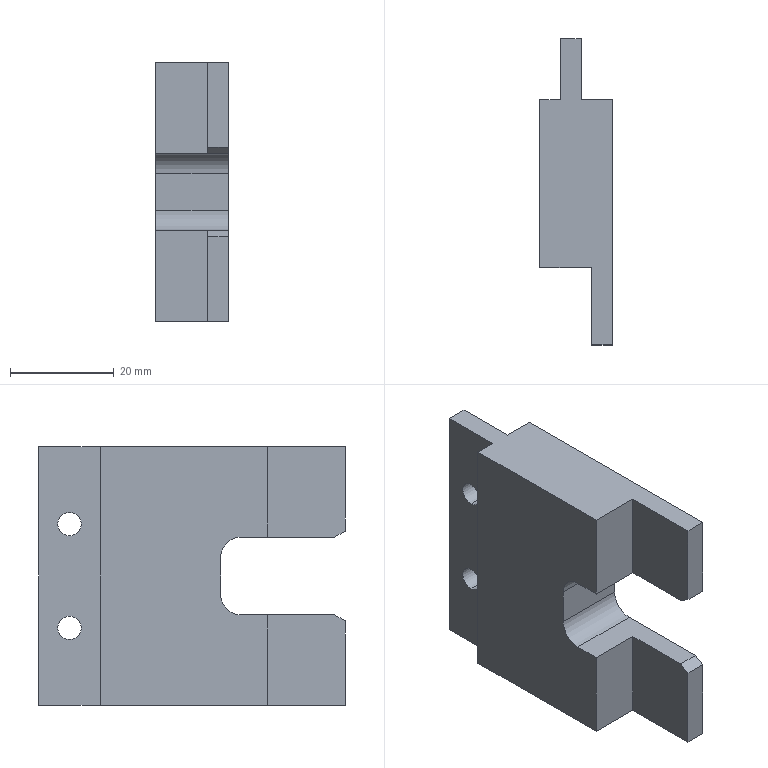Component | SolidWorks | WirePressingUnitLocatingPlate-1 | 1 solid | 26 faces | box 14 x 59 x 49.8 mm | volume 24958 mm3 | plane 20 | cylinder 6 | commonest cylinder face diameters 4.5 x4 8 x2
build123d program:
from build123d import *
from OCP.BRepFilletAPI import BRepFilletAPI_MakeChamfer

# Parameters (mm, degrees)
BOSS_EXTRUDE1_DEPTH = 14
SKETCH2_W           = 49.8
SKETCH2_H           = 11.8
CUT_EXTRUDE1_DEPTH  = 4
SKETCH4_W           = 45.507
SKETCH4_H           = 8.951
BOSS_EXTRUDE2_DEPTH = 10
SKETCH5_R           = 2.25
CUT_EXTRUDE3_DEPTH  = 10
SKETCH6_W           = 10
SKETCH6_H           = 15
SKETCH6_W_2         = 6
SKETCH6_H_2         = 11.8
CUT_EXTRUDE4_DEPTH  = 79.467
FILLET1_R           = 4
CHAMFER1_SIZE       = 2
CHAMFER1_SIZE2      = 1.155


with BuildPart() as part:
    # Sketch1 → Boss-Extrude1 (new body)
    with BuildSketch(Plane.XY):
        Polygon((-24.9, 0), (-7.5, 0), (-7.5, 24), (7.5, 24), (7.5, 0), (24.9, 0), (24.9, 59), (-24.9, 59), align=None)
    extrude(amount=BOSS_EXTRUDE1_DEPTH)

    # Sketch2 → Cut-Extrude1 (cut)
    with BuildSketch(Plane.XY.offset(14)):
        with Locations((0, 53.1)):
            Rectangle(SKETCH2_W, SKETCH2_H)
    extrude(amount=-CUT_EXTRUDE1_DEPTH, mode=Mode.SUBTRACT)

    # Sketch4 → Boss-Extrude2 (add)
    with BuildSketch(Plane(origin=(0, 0, 0), x_dir=(-1, 0, 0), z_dir=(0, 0, -1))):
        with Locations((-0.1161, 35.176)):
            Rectangle(SKETCH4_W, SKETCH4_H)
    extrude(amount=-BOSS_EXTRUDE2_DEPTH)

    # Sketch5 → Cut-Extrude3 (cut)
    with BuildSketch(Plane(origin=(0, 0, 0), x_dir=(-1, 0, 0), z_dir=(0, 0, -1))):
        with Locations((-10, 53.1)):
            Circle(SKETCH5_R)
        with Locations((10, 53.1)):
            Circle(SKETCH5_R)
    extrude(amount=-CUT_EXTRUDE3_DEPTH, mode=Mode.SUBTRACT)

    # Sketch6 → Cut-Extrude4 (cut, through all)
    with BuildSketch(Plane(origin=(24.9, 0, 0), x_dir=(0, 0, -1), z_dir=(1, 0, 0))):
        with Locations((-9, 7.5)):
            Rectangle(SKETCH6_W, SKETCH6_H)
        with Locations((-3, 53.1)):
            Rectangle(SKETCH6_W_2, SKETCH6_H_2)
    extrude(amount=-CUT_EXTRUDE4_DEPTH, mode=Mode.SUBTRACT)

    # Fillet1
    fillet1_edges = [part.edges().sort_by_distance(p)[0] for p in [
        (-7.5, 24, 7),
        (7.5, 24, 7),
    ]]
    fillet(fillet1_edges, radius=FILLET1_R)

    # Chamfer1: one chamfer whose edges measure the first distance from different faces: ONE call of the kernel's chamfer builder (chamfer() names one face for all edges)
    chamfer1_edges_1 = [part.edges().sort_by_distance(p)[0] for p in [
        (-7.5, 0, 2),
    ]]
    chamfer1_side_1 = [part.faces().sort_by_distance(p)[0] for p in [
        (-7.5, 10, 0.2441),
    ]]
    chamfer1_edges_2 = [part.edges().sort_by_distance(p)[0] for p in [
        (7.5, 0, 2),
    ]]
    chamfer1_side_2 = [part.faces().sort_by_distance(p)[0] for p in [
        (7.5, 10, 0.2441),
    ]]
    chamfer1 = BRepFilletAPI_MakeChamfer(part.part.solid().wrapped)
    for e in chamfer1_edges_1:
        chamfer1.Add(CHAMFER1_SIZE, CHAMFER1_SIZE2, e.wrapped, chamfer1_side_1[0].wrapped)  # the first distance lies on this face
    for e in chamfer1_edges_2:
        chamfer1.Add(CHAMFER1_SIZE, CHAMFER1_SIZE2, e.wrapped, chamfer1_side_2[0].wrapped)  # the first distance lies on this face
    add(Compound.cast(chamfer1.Shape()), mode=Mode.REPLACE)


solid = part.part

# Placed as in the assembly
solid = solid.moved(Location((14.565, -19.832, -145.015), (0, -90, 0)))
STEP:
#1=CARTESIAN_POINT('',(0.1797,1.31,-6.014));
#2=VERTEX_POINT('',#1);
#3=CARTESIAN_POINT('',(0.1797,1.31,-6.192));
#4=VERTEX_POINT('',#3);
#5=CARTESIAN_POINT('',(0.1797,1.31,-6.103));
#6=DIRECTION('',(1.,0.,-0.));
#7=DIRECTION('',(-0.,0.,-1.));
#8=AXIS2_PLACEMENT_3D('',#5,#6,#7);
#9=CIRCLE('',#8,0.08858);
#10=EDGE_CURVE('',#2,#4,#9,.T.);
#11=ORIENTED_EDGE('',*,*,#10,.F.);
#12=CARTESIAN_POINT('',(0.3372,1.31,-6.014));
#13=VERTEX_POINT('',#12);
#14=CARTESIAN_POINT('',(0.1797,1.31,-6.014));
#15=DIRECTION('',(1.,0.,-0.));
#16=VECTOR('',#15,39.37);
#17=LINE('',#14,#16);
#18=EDGE_CURVE('',#2,#13,#17,.T.);
#19=ORIENTED_EDGE('',*,*,#18,.T.);
#20=CARTESIAN_POINT('',(0.3372,1.31,-6.192));
#21=VERTEX_POINT('',#20);
#22=CARTESIAN_POINT('',(0.3372,1.31,-6.103));
#23=DIRECTION('',(1.,0.,-0.));
#24=DIRECTION('',(0.,-1.,0.));
#25=AXIS2_PLACEMENT_3D('',#22,#23,#24);
#26=CIRCLE('',#25,0.08858);
#27=EDGE_CURVE('',#13,#21,#26,.T.);
#28=ORIENTED_EDGE('',*,*,#27,.T.);
#29=CARTESIAN_POINT('',(0.1797,1.31,-6.192));
#30=DIRECTION('',(1.,0.,-0.));
#31=VECTOR('',#30,39.37);
#32=LINE('',#29,#31);
#33=EDGE_CURVE('',#4,#21,#32,.T.);
#34=ORIENTED_EDGE('',*,*,#33,.F.);
#35=EDGE_LOOP('',(#11,#19,#28,#34));
#36=FACE_OUTER_BOUND('',#35,.T.);
#37=CARTESIAN_POINT('',(0.1797,1.31,-6.103));
#38=DIRECTION('',(1.,0.,-0.));
#39=DIRECTION('',(-0.,0.,-1.));
#40=AXIS2_PLACEMENT_3D('',#37,#38,#39);
#41=CYLINDRICAL_SURFACE('',#40,0.08858);
#42=ADVANCED_FACE('',(#36),#41,.F.);
#43=CARTESIAN_POINT('',(0.1797,1.31,-5.227));
#44=VERTEX_POINT('',#43);
#45=CARTESIAN_POINT('',(0.1797,1.31,-5.404));
#46=VERTEX_POINT('',#45);
#47=CARTESIAN_POINT('',(0.1797,1.31,-5.316));
#48=DIRECTION('',(1.,0.,-0.));
#49=DIRECTION('',(-0.,0.,-1.));
#50=AXIS2_PLACEMENT_3D('',#47,#48,#49);
#51=CIRCLE('',#50,0.08858);
#52=EDGE_CURVE('',#44,#46,#51,.T.);
#53=ORIENTED_EDGE('',*,*,#52,.F.);
#54=CARTESIAN_POINT('',(0.3372,1.31,-5.227));
#55=VERTEX_POINT('',#54);
#56=CARTESIAN_POINT('',(0.1797,1.31,-5.227));
#57=DIRECTION('',(1.,0.,-0.));
#58=VECTOR('',#57,39.37);
#59=LINE('',#56,#58);
#60=EDGE_CURVE('',#44,#55,#59,.T.);
#61=ORIENTED_EDGE('',*,*,#60,.T.);
#62=CARTESIAN_POINT('',(0.3372,1.31,-5.404));
#63=VERTEX_POINT('',#62);
#64=CARTESIAN_POINT('',(0.3372,1.31,-5.316));
#65=DIRECTION('',(1.,0.,-0.));
#66=DIRECTION('',(0.,-1.,0.));
#67=AXIS2_PLACEMENT_3D('',#64,#65,#66);
#68=CIRCLE('',#67,0.08858);
#69=EDGE_CURVE('',#55,#63,#68,.T.);
#70=ORIENTED_EDGE('',*,*,#69,.T.);
#71=CARTESIAN_POINT('',(0.1797,1.31,-5.404));
#72=DIRECTION('',(1.,0.,-0.));
#73=VECTOR('',#72,39.37);
#74=LINE('',#71,#73);
#75=EDGE_CURVE('',#46,#63,#74,.T.);
#76=ORIENTED_EDGE('',*,*,#75,.F.);
#77=EDGE_LOOP('',(#53,#61,#70,#76));
#78=FACE_OUTER_BOUND('',#77,.T.);
#79=CARTESIAN_POINT('',(0.1797,1.31,-5.316));
#80=DIRECTION('',(1.,0.,-0.));
#81=DIRECTION('',(-0.,0.,-1.));
#82=AXIS2_PLACEMENT_3D('',#79,#80,#81);
#83=CYLINDRICAL_SURFACE('',#82,0.08858);
#84=ADVANCED_FACE('',(#78),#83,.F.);
#85=CARTESIAN_POINT('',(0.1797,1.542,-4.729));
#86=VERTEX_POINT('',#85);
#87=CARTESIAN_POINT('',(0.3372,1.542,-4.729));
#88=VERTEX_POINT('',#87);
#89=CARTESIAN_POINT('',(0.02224,1.542,-4.729));
#90=DIRECTION('',(1.,0.,-0.));
#91=VECTOR('',#90,39.37);
#92=LINE('',#89,#91);
#93=EDGE_CURVE('',#86,#88,#92,.T.);
#94=ORIENTED_EDGE('',*,*,#93,.T.);
#95=CARTESIAN_POINT('',(0.3372,1.542,-6.69));
#96=VERTEX_POINT('',#95);
#97=CARTESIAN_POINT('',(0.3372,1.542,-6.69));
#98=DIRECTION('',(0.,0.,1.));
#99=VECTOR('',#98,39.37);
#100=LINE('',#97,#99);
#101=EDGE_CURVE('',#96,#88,#100,.T.);
#102=ORIENTED_EDGE('',*,*,#101,.F.);
#103=CARTESIAN_POINT('',(0.1797,1.542,-6.69));
#104=VERTEX_POINT('',#103);
#105=CARTESIAN_POINT('',(0.02224,1.542,-6.69));
#106=DIRECTION('',(1.,0.,-0.));
#107=VECTOR('',#106,39.37);
#108=LINE('',#105,#107);
#109=EDGE_CURVE('',#104,#96,#108,.T.);
#110=ORIENTED_EDGE('',*,*,#109,.F.);
#111=CARTESIAN_POINT('',(0.1797,1.542,-6.69));
#112=DIRECTION('',(-0.,0.,-1.));
#113=VECTOR('',#112,39.37);
#114=LINE('',#111,#113);
#115=EDGE_CURVE('',#86,#104,#114,.T.);
#116=ORIENTED_EDGE('',*,*,#115,.F.);
#117=EDGE_LOOP('',(#94,#102,#110,#116));
#118=FACE_OUTER_BOUND('',#117,.T.);
#119=CARTESIAN_POINT('',(0.02224,1.542,-4.729));
#120=DIRECTION('',(0.,-1.,0.));
#121=DIRECTION('',(1.,0.,-0.));
#122=AXIS2_PLACEMENT_3D('',#119,#120,#121);
#123=PLANE('',#122);
#124=ADVANCED_FACE('',(#118),#123,.F.);
#125=CARTESIAN_POINT('',(0.02224,0.1641,-5.847));
#126=VERTEX_POINT('',#125);
#127=CARTESIAN_POINT('',(0.02224,0.1641,-5.571));
#128=VERTEX_POINT('',#127);
#129=CARTESIAN_POINT('',(0.02224,0.1641,-6.005));
#130=DIRECTION('',(0.,0.,1.));
#131=VECTOR('',#130,39.37);
#132=LINE('',#129,#131);
#133=EDGE_CURVE('',#126,#128,#132,.T.);
#134=ORIENTED_EDGE('',*,*,#133,.F.);
#135=CARTESIAN_POINT('',(0.5734,0.1641,-5.847));
#136=VERTEX_POINT('',#135);
#137=CARTESIAN_POINT('',(0.5734,0.1641,-5.847));
#138=DIRECTION('',(1.,0.,-0.));
#139=VECTOR('',#138,39.37);
#140=LINE('',#137,#139);
#141=EDGE_CURVE('',#126,#136,#140,.T.);
#142=ORIENTED_EDGE('',*,*,#141,.T.);
#143=CARTESIAN_POINT('',(0.5734,0.1641,-5.571));
#144=VERTEX_POINT('',#143);
#145=CARTESIAN_POINT('',(0.5734,0.1641,-6.005));
#146=DIRECTION('',(0.,0.,1.));
#147=VECTOR('',#146,39.37);
#148=LINE('',#145,#147);
#149=EDGE_CURVE('',#136,#144,#148,.T.);
#150=ORIENTED_EDGE('',*,*,#149,.T.);
#151=CARTESIAN_POINT('',(0.02224,0.1641,-5.571));
#152=DIRECTION('',(-1.,0.,0.));
#153=VECTOR('',#152,39.37);
#154=LINE('',#151,#153);
#155=EDGE_CURVE('',#144,#128,#154,.T.);
#156=ORIENTED_EDGE('',*,*,#155,.T.);
#157=EDGE_LOOP('',(#134,#142,#150,#156));
#158=FACE_OUTER_BOUND('',#157,.T.);
#159=CARTESIAN_POINT('',(0.02224,0.1641,-6.005));
#160=DIRECTION('',(0.,1.,0.));
#161=DIRECTION('',(-1.,0.,0.));
#162=AXIS2_PLACEMENT_3D('',#159,#160,#161);
#163=PLANE('',#162);
#164=ADVANCED_FACE('',(#158),#163,.F.);
#165=CARTESIAN_POINT('',(0.5734,0.006624,-5.414));
#166=VERTEX_POINT('',#165);
#167=CARTESIAN_POINT('',(0.5734,-0.702,-5.414));
#168=VERTEX_POINT('',#167);
#169=CARTESIAN_POINT('',(0.5734,0.1641,-5.414));
#170=DIRECTION('',(0.,-1.,0.));
#171=VECTOR('',#170,39.37);
#172=LINE('',#169,#171);
#173=EDGE_CURVE('',#166,#168,#172,.T.);
#174=ORIENTED_EDGE('',*,*,#173,.T.);
#175=CARTESIAN_POINT('',(0.4159,-0.702,-5.414));
#176=VERTEX_POINT('',#175);
#177=CARTESIAN_POINT('',(0.02224,-0.702,-5.414));
#178=DIRECTION('',(-1.,0.,0.));
#179=VECTOR('',#178,39.37);
#180=LINE('',#177,#179);
#181=EDGE_CURVE('',#168,#176,#180,.T.);
#182=ORIENTED_EDGE('',*,*,#181,.T.);
#183=CARTESIAN_POINT('',(0.4159,-0.1902,-5.414));
#184=VERTEX_POINT('',#183);
#185=CARTESIAN_POINT('',(0.4159,0.1641,-5.414));
#186=DIRECTION('',(-0.,1.,-0.));
#187=VECTOR('',#186,39.37);
#188=LINE('',#185,#187);
#189=EDGE_CURVE('',#176,#184,#188,.T.);
#190=ORIENTED_EDGE('',*,*,#189,.T.);
#191=CARTESIAN_POINT('',(0.02224,-0.1902,-5.414));
#192=VERTEX_POINT('',#191);
#193=CARTESIAN_POINT('',(0.02224,-0.1902,-5.414));
#194=DIRECTION('',(-1.,0.,0.));
#195=VECTOR('',#194,39.37);
#196=LINE('',#193,#195);
#197=EDGE_CURVE('',#184,#192,#196,.T.);
#198=ORIENTED_EDGE('',*,*,#197,.T.);
#199=CARTESIAN_POINT('',(0.02224,0.006624,-5.414));
#200=VERTEX_POINT('',#199);
#201=CARTESIAN_POINT('',(0.02224,0.1641,-5.414));
#202=DIRECTION('',(0.,-1.,0.));
#203=VECTOR('',#202,39.37);
#204=LINE('',#201,#203);
#205=EDGE_CURVE('',#200,#192,#204,.T.);
#206=ORIENTED_EDGE('',*,*,#205,.F.);
#207=CARTESIAN_POINT('',(0.5734,0.006624,-5.414));
#208=DIRECTION('',(1.,0.,-0.));
#209=VECTOR('',#208,39.37);
#210=LINE('',#207,#209);
#211=EDGE_CURVE('',#200,#166,#210,.T.);
#212=ORIENTED_EDGE('',*,*,#211,.T.);
#213=EDGE_LOOP('',(#174,#182,#190,#198,#206,#212));
#214=FACE_OUTER_BOUND('',#213,.T.);
#215=CARTESIAN_POINT('',(0.02224,0.1641,-5.414));
#216=DIRECTION('',(0.,0.,1.));
#217=DIRECTION('',(-0.,1.,-0.));
#218=AXIS2_PLACEMENT_3D('',#215,#216,#217);
#219=PLANE('',#218);
#220=ADVANCED_FACE('',(#214),#219,.F.);
#221=CARTESIAN_POINT('',(0.4159,-0.7808,-5.369));
#222=VERTEX_POINT('',#221);
#223=CARTESIAN_POINT('',(0.4159,-0.7808,-4.729));
#224=VERTEX_POINT('',#223);
#225=CARTESIAN_POINT('',(0.4159,-0.7808,-6.69));
#226=DIRECTION('',(0.,0.,1.));
#227=VECTOR('',#226,39.37);
#228=LINE('',#225,#227);
#229=EDGE_CURVE('',#222,#224,#228,.T.);
#230=ORIENTED_EDGE('',*,*,#229,.F.);
#231=CARTESIAN_POINT('',(0.5734,-0.7808,-5.369));
#232=VERTEX_POINT('',#231);
#233=CARTESIAN_POINT('',(0.02224,-0.7808,-5.369));
#234=DIRECTION('',(1.,0.,-0.));
#235=VECTOR('',#234,39.37);
#236=LINE('',#233,#235);
#237=EDGE_CURVE('',#222,#232,#236,.T.);
#238=ORIENTED_EDGE('',*,*,#237,.T.);
#239=CARTESIAN_POINT('',(0.5734,-0.7808,-4.729));
#240=VERTEX_POINT('',#239);
#241=CARTESIAN_POINT('',(0.5734,-0.7808,-5.414));
#242=DIRECTION('',(0.,0.,1.));
#243=VECTOR('',#242,39.37);
#244=LINE('',#241,#243);
#245=EDGE_CURVE('',#232,#240,#244,.T.);
#246=ORIENTED_EDGE('',*,*,#245,.T.);
#247=CARTESIAN_POINT('',(0.02224,-0.7808,-4.729));
#248=DIRECTION('',(1.,0.,-0.));
#249=VECTOR('',#248,39.37);
#250=LINE('',#247,#249);
#251=EDGE_CURVE('',#224,#240,#250,.T.);
#252=ORIENTED_EDGE('',*,*,#251,.F.);
#253=EDGE_LOOP('',(#230,#238,#246,#252));
#254=FACE_OUTER_BOUND('',#253,.T.);
#255=CARTESIAN_POINT('',(0.02224,-0.7808,-5.414));
#256=DIRECTION('',(0.,1.,0.));
#257=DIRECTION('',(-1.,0.,0.));
#258=AXIS2_PLACEMENT_3D('',#255,#256,#257);
#259=PLANE('',#258);
#260=ADVANCED_FACE('',(#254),#259,.F.);
#261=CARTESIAN_POINT('',(0.3372,1.077,-4.729));
#262=VERTEX_POINT('',#261);
#263=CARTESIAN_POINT('',(0.5734,1.077,-4.729));
#264=VERTEX_POINT('',#263);
#265=CARTESIAN_POINT('',(0.3372,1.077,-4.729));
#266=DIRECTION('',(1.,0.,-0.));
#267=VECTOR('',#266,39.37);
#268=LINE('',#265,#267);
#269=EDGE_CURVE('',#262,#264,#268,.T.);
#270=ORIENTED_EDGE('',*,*,#269,.F.);
#271=CARTESIAN_POINT('',(0.3372,1.542,-4.729));
#272=DIRECTION('',(0.,-1.,-0.));
#273=VECTOR('',#272,39.37);
#274=LINE('',#271,#273);
#275=EDGE_CURVE('',#88,#262,#274,.T.);
#276=ORIENTED_EDGE('',*,*,#275,.F.);
#277=ORIENTED_EDGE('',*,*,#93,.F.);
#278=CARTESIAN_POINT('',(0.1797,1.077,-4.729));
#279=VERTEX_POINT('',#278);
#280=CARTESIAN_POINT('',(0.1797,1.542,-4.729));
#281=DIRECTION('',(0.,1.,0.));
#282=VECTOR('',#281,39.37);
#283=LINE('',#280,#282);
#284=EDGE_CURVE('',#279,#86,#283,.T.);
#285=ORIENTED_EDGE('',*,*,#284,.F.);
#286=CARTESIAN_POINT('',(0.02224,1.077,-4.729));
#287=VERTEX_POINT('',#286);
#288=CARTESIAN_POINT('',(0.1797,1.077,-4.729));
#289=DIRECTION('',(-1.,0.,0.));
#290=VECTOR('',#289,39.37);
#291=LINE('',#288,#290);
#292=EDGE_CURVE('',#279,#287,#291,.T.);
#293=ORIENTED_EDGE('',*,*,#292,.T.);
#294=CARTESIAN_POINT('',(0.02224,-0.1902,-4.729));
#295=VERTEX_POINT('',#294);
#296=CARTESIAN_POINT('',(0.02224,-0.7808,-4.729));
#297=DIRECTION('',(0.,1.,0.));
#298=VECTOR('',#297,39.37);
#299=LINE('',#296,#298);
#300=EDGE_CURVE('',#295,#287,#299,.T.);
#301=ORIENTED_EDGE('',*,*,#300,.F.);
#302=CARTESIAN_POINT('',(0.4159,-0.1902,-4.729));
#303=VERTEX_POINT('',#302);
#304=CARTESIAN_POINT('',(0.02224,-0.1902,-4.729));
#305=DIRECTION('',(-1.,0.,0.));
#306=VECTOR('',#305,39.37);
#307=LINE('',#304,#306);
#308=EDGE_CURVE('',#303,#295,#307,.T.);
#309=ORIENTED_EDGE('',*,*,#308,.F.);
#310=CARTESIAN_POINT('',(0.4159,-0.1902,-4.729));
#311=DIRECTION('',(-0.,1.,0.));
#312=VECTOR('',#311,39.37);
#313=LINE('',#310,#312);
#314=EDGE_CURVE('',#224,#303,#313,.T.);
#315=ORIENTED_EDGE('',*,*,#314,.F.);
#316=ORIENTED_EDGE('',*,*,#251,.T.);
#317=CARTESIAN_POINT('',(0.5734,-0.7808,-4.729));
#318=DIRECTION('',(0.,1.,0.));
#319=VECTOR('',#318,39.37);
#320=LINE('',#317,#319);
#321=EDGE_CURVE('',#240,#264,#320,.T.);
#322=ORIENTED_EDGE('',*,*,#321,.T.);
#323=EDGE_LOOP('',(#270,#276,#277,#285,#293,#301,#309,#315,#316,#322));
#324=FACE_OUTER_BOUND('',#323,.T.);
#325=CARTESIAN_POINT('',(0.02224,-0.7808,-4.729));
#326=DIRECTION('',(-0.,0.,-1.));
#327=DIRECTION('',(-1.,0.,0.));
#328=AXIS2_PLACEMENT_3D('',#325,#326,#327);
#329=PLANE('',#328);
#330=ADVANCED_FACE('',(#324),#329,.F.);
#331=ORIENTED_EDGE('',*,*,#109,.T.);
#332=CARTESIAN_POINT('',(0.3372,1.077,-6.69));
#333=VERTEX_POINT('',#332);
#334=CARTESIAN_POINT('',(0.3372,1.542,-6.69));
#335=DIRECTION('',(0.,-1.,-0.));
#336=VECTOR('',#335,39.37);
#337=LINE('',#334,#336);
#338=EDGE_CURVE('',#96,#333,#337,.T.);
#339=ORIENTED_EDGE('',*,*,#338,.T.);
#340=CARTESIAN_POINT('',(0.5734,1.077,-6.69));
#341=VERTEX_POINT('',#340);
#342=CARTESIAN_POINT('',(0.3372,1.077,-6.69));
#343=DIRECTION('',(1.,0.,-0.));
#344=VECTOR('',#343,39.37);
#345=LINE('',#342,#344);
#346=EDGE_CURVE('',#333,#341,#345,.T.);
#347=ORIENTED_EDGE('',*,*,#346,.T.);
#348=CARTESIAN_POINT('',(0.5734,-0.7808,-6.69));
#349=VERTEX_POINT('',#348);
#350=CARTESIAN_POINT('',(0.5734,-0.7808,-6.69));
#351=DIRECTION('',(0.,-1.,0.));
#352=VECTOR('',#351,39.37);
#353=LINE('',#350,#352);
#354=EDGE_CURVE('',#341,#349,#353,.T.);
#355=ORIENTED_EDGE('',*,*,#354,.T.);
#356=CARTESIAN_POINT('',(0.4159,-0.7808,-6.69));
#357=VERTEX_POINT('',#356);
#358=CARTESIAN_POINT('',(0.02224,-0.7808,-6.69));
#359=DIRECTION('',(1.,0.,-0.));
#360=VECTOR('',#359,39.37);
#361=LINE('',#358,#360);
#362=EDGE_CURVE('',#357,#349,#361,.T.);
#363=ORIENTED_EDGE('',*,*,#362,.F.);
#364=CARTESIAN_POINT('',(0.4159,-0.1902,-6.69));
#365=VERTEX_POINT('',#364);
#366=CARTESIAN_POINT('',(0.4159,-0.1902,-6.69));
#367=DIRECTION('',(-0.,1.,0.));
#368=VECTOR('',#367,39.37);
#369=LINE('',#366,#368);
#370=EDGE_CURVE('',#357,#365,#369,.T.);
#371=ORIENTED_EDGE('',*,*,#370,.T.);
#372=CARTESIAN_POINT('',(0.02224,-0.1902,-6.69));
#373=VERTEX_POINT('',#372);
#374=CARTESIAN_POINT('',(0.02224,-0.1902,-6.69));
#375=DIRECTION('',(-1.,0.,0.));
#376=VECTOR('',#375,39.37);
#377=LINE('',#374,#376);
#378=EDGE_CURVE('',#365,#373,#377,.T.);
#379=ORIENTED_EDGE('',*,*,#378,.T.);
#380=CARTESIAN_POINT('',(0.02224,1.077,-6.69));
#381=VERTEX_POINT('',#380);
#382=CARTESIAN_POINT('',(0.02224,-0.7808,-6.69));
#383=DIRECTION('',(0.,-1.,0.));
#384=VECTOR('',#383,39.37);
#385=LINE('',#382,#384);
#386=EDGE_CURVE('',#381,#373,#385,.T.);
#387=ORIENTED_EDGE('',*,*,#386,.F.);
#388=CARTESIAN_POINT('',(0.1797,1.077,-6.69));
#389=VERTEX_POINT('',#388);
#390=CARTESIAN_POINT('',(0.1797,1.077,-6.69));
#391=DIRECTION('',(-1.,0.,0.));
#392=VECTOR('',#391,39.37);
#393=LINE('',#390,#392);
#394=EDGE_CURVE('',#389,#381,#393,.T.);
#395=ORIENTED_EDGE('',*,*,#394,.F.);
#396=CARTESIAN_POINT('',(0.1797,1.542,-6.69));
#397=DIRECTION('',(0.,-1.,0.));
#398=VECTOR('',#397,39.37);
#399=LINE('',#396,#398);
#400=EDGE_CURVE('',#104,#389,#399,.T.);
#401=ORIENTED_EDGE('',*,*,#400,.F.);
#402=EDGE_LOOP('',(#331,#339,#347,#355,#363,#371,#379,#387,#395,#401));
#403=FACE_OUTER_BOUND('',#402,.T.);
#404=CARTESIAN_POINT('',(0.02224,-0.7808,-6.69));
#405=DIRECTION('',(0.,0.,1.));
#406=DIRECTION('',(1.,0.,-0.));
#407=AXIS2_PLACEMENT_3D('',#404,#405,#406);
#408=PLANE('',#407);
#409=ADVANCED_FACE('',(#403),#408,.F.);
#410=CARTESIAN_POINT('',(0.5734,-0.7808,-6.05));
#411=VERTEX_POINT('',#410);
#412=CARTESIAN_POINT('',(0.5734,-0.7808,-6.69));
#413=DIRECTION('',(0.,0.,1.));
#414=VECTOR('',#413,39.37);
#415=LINE('',#412,#414);
#416=EDGE_CURVE('',#349,#411,#415,.T.);
#417=ORIENTED_EDGE('',*,*,#416,.T.);
#418=CARTESIAN_POINT('',(0.4159,-0.7808,-6.05));
#419=VERTEX_POINT('',#418);
#420=CARTESIAN_POINT('',(0.02224,-0.7808,-6.05));
#421=DIRECTION('',(-1.,0.,0.));
#422=VECTOR('',#421,39.37);
#423=LINE('',#420,#422);
#424=EDGE_CURVE('',#411,#419,#423,.T.);
#425=ORIENTED_EDGE('',*,*,#424,.T.);
#426=CARTESIAN_POINT('',(0.4159,-0.7808,-6.69));
#427=DIRECTION('',(0.,0.,1.));
#428=VECTOR('',#427,39.37);
#429=LINE('',#426,#428);
#430=EDGE_CURVE('',#357,#419,#429,.T.);
#431=ORIENTED_EDGE('',*,*,#430,.F.);
#432=ORIENTED_EDGE('',*,*,#362,.T.);
#433=EDGE_LOOP('',(#417,#425,#431,#432));
#434=FACE_OUTER_BOUND('',#433,.T.);
#435=CARTESIAN_POINT('',(0.02224,-0.7808,-6.69));
#436=DIRECTION('',(0.,1.,0.));
#437=DIRECTION('',(-1.,0.,0.));
#438=AXIS2_PLACEMENT_3D('',#435,#436,#437);
#439=PLANE('',#438);
#440=ADVANCED_FACE('',(#434),#439,.F.);
#441=CARTESIAN_POINT('',(0.4159,-0.1902,-6.005));
#442=VERTEX_POINT('',#441);
#443=CARTESIAN_POINT('',(0.4159,-0.702,-6.005));
#444=VERTEX_POINT('',#443);
#445=CARTESIAN_POINT('',(0.4159,-0.7808,-6.005));
#446=DIRECTION('',(0.,-1.,-0.));
#447=VECTOR('',#446,39.37);
#448=LINE('',#445,#447);
#449=EDGE_CURVE('',#442,#444,#448,.T.);
#450=ORIENTED_EDGE('',*,*,#449,.T.);
#451=CARTESIAN_POINT('',(0.5734,-0.702,-6.005));
#452=VERTEX_POINT('',#451);
#453=CARTESIAN_POINT('',(0.02224,-0.702,-6.005));
#454=DIRECTION('',(1.,0.,-0.));
#455=VECTOR('',#454,39.37);
#456=LINE('',#453,#455);
#457=EDGE_CURVE('',#444,#452,#456,.T.);
#458=ORIENTED_EDGE('',*,*,#457,.T.);
#459=CARTESIAN_POINT('',(0.5734,0.006624,-6.005));
#460=VERTEX_POINT('',#459);
#461=CARTESIAN_POINT('',(0.5734,-0.7808,-6.005));
#462=DIRECTION('',(0.,1.,0.));
#463=VECTOR('',#462,39.37);
#464=LINE('',#461,#463);
#465=EDGE_CURVE('',#452,#460,#464,.T.);
#466=ORIENTED_EDGE('',*,*,#465,.T.);
#467=CARTESIAN_POINT('',(0.02224,0.006624,-6.005));
#468=VERTEX_POINT('',#467);
#469=CARTESIAN_POINT('',(0.02224,0.006624,-6.005));
#470=DIRECTION('',(-1.,0.,0.));
#471=VECTOR('',#470,39.37);
#472=LINE('',#469,#471);
#473=EDGE_CURVE('',#460,#468,#472,.T.);
#474=ORIENTED_EDGE('',*,*,#473,.T.);
#475=CARTESIAN_POINT('',(0.02224,-0.1902,-6.005));
#476=VERTEX_POINT('',#475);
#477=CARTESIAN_POINT('',(0.02224,-0.7808,-6.005));
#478=DIRECTION('',(0.,1.,0.));
#479=VECTOR('',#478,39.37);
#480=LINE('',#477,#479);
#481=EDGE_CURVE('',#476,#468,#480,.T.);
#482=ORIENTED_EDGE('',*,*,#481,.F.);
#483=CARTESIAN_POINT('',(0.02224,-0.1902,-6.005));
#484=DIRECTION('',(1.,0.,-0.));
#485=VECTOR('',#484,39.37);
#486=LINE('',#483,#485);
#487=EDGE_CURVE('',#476,#442,#486,.T.);
#488=ORIENTED_EDGE('',*,*,#487,.T.);
#489=EDGE_LOOP('',(#450,#458,#466,#474,#482,#488));
#490=FACE_OUTER_BOUND('',#489,.T.);
#491=CARTESIAN_POINT('',(0.02224,-0.7808,-6.005));
#492=DIRECTION('',(-0.,0.,-1.));
#493=DIRECTION('',(-0.,-1.,-0.));
#494=AXIS2_PLACEMENT_3D('',#491,#492,#493);
#495=PLANE('',#494);
#496=ADVANCED_FACE('',(#490),#495,.F.);
#497=ORIENTED_EDGE('',*,*,#386,.T.);
#498=CARTESIAN_POINT('',(0.02224,-0.1902,-6.69));
#499=DIRECTION('',(0.,0.,1.));
#500=VECTOR('',#499,39.37);
#501=LINE('',#498,#500);
#502=EDGE_CURVE('',#373,#476,#501,.T.);
#503=ORIENTED_EDGE('',*,*,#502,.T.);
#504=ORIENTED_EDGE('',*,*,#481,.T.);
#505=CARTESIAN_POINT('',(0.02224,0.006624,-5.847));
#506=DIRECTION('',(1.,0.,-0.));
#507=DIRECTION('',(-0.,0.,-1.));
#508=AXIS2_PLACEMENT_3D('',#505,#506,#507);
#509=CIRCLE('',#508,0.1575);
#510=EDGE_CURVE('',#468,#126,#509,.T.);
#511=ORIENTED_EDGE('',*,*,#510,.T.);
#512=ORIENTED_EDGE('',*,*,#133,.T.);
#513=CARTESIAN_POINT('',(0.02224,0.006624,-5.571));
#514=DIRECTION('',(1.,0.,-0.));
#515=DIRECTION('',(-0.,0.,-1.));
#516=AXIS2_PLACEMENT_3D('',#513,#514,#515);
#517=CIRCLE('',#516,0.1575);
#518=EDGE_CURVE('',#128,#200,#517,.T.);
#519=ORIENTED_EDGE('',*,*,#518,.T.);
#520=ORIENTED_EDGE('',*,*,#205,.T.);
#521=CARTESIAN_POINT('',(0.02224,-0.1902,-5.414));
#522=DIRECTION('',(0.,0.,1.));
#523=VECTOR('',#522,39.37);
#524=LINE('',#521,#523);
#525=EDGE_CURVE('',#192,#295,#524,.T.);
#526=ORIENTED_EDGE('',*,*,#525,.T.);
#527=ORIENTED_EDGE('',*,*,#300,.T.);
#528=CARTESIAN_POINT('',(0.02224,1.077,-6.69));
#529=DIRECTION('',(0.,0.,1.));
#530=VECTOR('',#529,39.37);
#531=LINE('',#528,#530);
#532=EDGE_CURVE('',#381,#287,#531,.T.);
#533=ORIENTED_EDGE('',*,*,#532,.F.);
#534=EDGE_LOOP('',(#497,#503,#504,#511,#512,#519,#520,#526,#527,#533));
#535=FACE_OUTER_BOUND('',#534,.T.);
#536=CARTESIAN_POINT('',(0.02224,0.1641,-5.414));
#537=DIRECTION('',(1.,0.,-0.));
#538=DIRECTION('',(-0.,0.,-1.));
#539=AXIS2_PLACEMENT_3D('',#536,#537,#538);
#540=PLANE('',#539);
#541=ADVANCED_FACE('',(#535),#540,.F.);
#542=ORIENTED_EDGE('',*,*,#465,.F.);
#543=CARTESIAN_POINT('',(0.5734,0.2033,-5.482));
#544=DIRECTION('',(-0.,-0.866,-0.5));
#545=VECTOR('',#544,39.37);
#546=LINE('',#543,#545);
#547=EDGE_CURVE('',#452,#411,#546,.T.);
#548=ORIENTED_EDGE('',*,*,#547,.T.);
#549=ORIENTED_EDGE('',*,*,#416,.F.);
#550=ORIENTED_EDGE('',*,*,#354,.F.);
#551=CARTESIAN_POINT('',(0.5734,1.077,-6.69));
#552=DIRECTION('',(0.,0.,1.));
#553=VECTOR('',#552,39.37);
#554=LINE('',#551,#553);
#555=EDGE_CURVE('',#341,#264,#554,.T.);
#556=ORIENTED_EDGE('',*,*,#555,.T.);
#557=ORIENTED_EDGE('',*,*,#321,.F.);
#558=ORIENTED_EDGE('',*,*,#245,.F.);
#559=CARTESIAN_POINT('',(0.5734,-0.05243,-5.789));
#560=DIRECTION('',(-0.,0.866,-0.5));
#561=VECTOR('',#560,39.37);
#562=LINE('',#559,#561);
#563=EDGE_CURVE('',#232,#168,#562,.T.);
#564=ORIENTED_EDGE('',*,*,#563,.T.);
#565=ORIENTED_EDGE('',*,*,#173,.F.);
#566=CARTESIAN_POINT('',(0.5734,0.006624,-5.571));
#567=DIRECTION('',(-1.,0.,0.));
#568=DIRECTION('',(-0.,0.,-1.));
#569=AXIS2_PLACEMENT_3D('',#566,#567,#568);
#570=CIRCLE('',#569,0.1575);
#571=EDGE_CURVE('',#166,#144,#570,.T.);
#572=ORIENTED_EDGE('',*,*,#571,.T.);
#573=ORIENTED_EDGE('',*,*,#149,.F.);
#574=CARTESIAN_POINT('',(0.5734,0.006624,-5.847));
#575=DIRECTION('',(-1.,0.,0.));
#576=DIRECTION('',(-0.,0.,-1.));
#577=AXIS2_PLACEMENT_3D('',#574,#575,#576);
#578=CIRCLE('',#577,0.1575);
#579=EDGE_CURVE('',#136,#460,#578,.T.);
#580=ORIENTED_EDGE('',*,*,#579,.T.);
#581=EDGE_LOOP('',(#542,#548,#549,#550,#556,#557,#558,#564,#565,#572,#573,#580));
#582=FACE_OUTER_BOUND('',#581,.T.);
#583=CARTESIAN_POINT('',(0.5734,0.1641,-5.414));
#584=DIRECTION('',(1.,0.,-0.));
#585=DIRECTION('',(-0.,0.,-1.));
#586=AXIS2_PLACEMENT_3D('',#583,#584,#585);
#587=PLANE('',#586);
#588=ADVANCED_FACE('',(#582),#587,.T.);
#589=ORIENTED_EDGE('',*,*,#532,.T.);
#590=ORIENTED_EDGE('',*,*,#292,.F.);
#591=CARTESIAN_POINT('',(0.1797,1.077,-6.69));
#592=DIRECTION('',(0.,0.,1.));
#593=VECTOR('',#592,39.37);
#594=LINE('',#591,#593);
#595=EDGE_CURVE('',#389,#279,#594,.T.);
#596=ORIENTED_EDGE('',*,*,#595,.F.);
#597=ORIENTED_EDGE('',*,*,#394,.T.);
#598=EDGE_LOOP('',(#589,#590,#596,#597));
#599=FACE_OUTER_BOUND('',#598,.T.);
#600=CARTESIAN_POINT('',(0.1797,1.077,-6.69));
#601=DIRECTION('',(0.,-1.,0.));
#602=DIRECTION('',(1.,0.,-0.));
#603=AXIS2_PLACEMENT_3D('',#600,#601,#602);
#604=PLANE('',#603);
#605=ADVANCED_FACE('',(#599),#604,.F.);
#606=CARTESIAN_POINT('',(0.1797,1.31,-6.103));
#607=DIRECTION('',(1.,0.,-0.));
#608=DIRECTION('',(-0.,0.,-1.));
#609=AXIS2_PLACEMENT_3D('',#606,#607,#608);
#610=CIRCLE('',#609,0.08858);
#611=EDGE_CURVE('',#4,#2,#610,.T.);
#612=ORIENTED_EDGE('',*,*,#611,.T.);
#613=ORIENTED_EDGE('',*,*,#10,.T.);
#614=EDGE_LOOP('',(#612,#613));
#615=FACE_BOUND('',#614,.T.);
#616=CARTESIAN_POINT('',(0.1797,1.31,-5.316));
#617=DIRECTION('',(1.,0.,-0.));
#618=DIRECTION('',(-0.,0.,-1.));
#619=AXIS2_PLACEMENT_3D('',#616,#617,#618);
#620=CIRCLE('',#619,0.08858);
#621=EDGE_CURVE('',#46,#44,#620,.T.);
#622=ORIENTED_EDGE('',*,*,#621,.T.);
#623=ORIENTED_EDGE('',*,*,#52,.T.);
#624=EDGE_LOOP('',(#622,#623));
#625=FACE_BOUND('',#624,.T.);
#626=ORIENTED_EDGE('',*,*,#400,.T.);
#627=ORIENTED_EDGE('',*,*,#595,.T.);
#628=ORIENTED_EDGE('',*,*,#284,.T.);
#629=ORIENTED_EDGE('',*,*,#115,.T.);
#630=EDGE_LOOP('',(#626,#627,#628,#629));
#631=FACE_OUTER_BOUND('',#630,.T.);
#632=CARTESIAN_POINT('',(0.1797,1.077,-6.69));
#633=DIRECTION('',(-1.,0.,0.));
#634=DIRECTION('',(0.,0.,1.));
#635=AXIS2_PLACEMENT_3D('',#632,#633,#634);
#636=PLANE('',#635);
#637=ADVANCED_FACE('',(#615,#625,#631),#636,.T.);
#638=ORIENTED_EDGE('',*,*,#60,.F.);
#639=ORIENTED_EDGE('',*,*,#621,.F.);
#640=ORIENTED_EDGE('',*,*,#75,.T.);
#641=CARTESIAN_POINT('',(0.3372,1.31,-5.316));
#642=DIRECTION('',(1.,0.,-0.));
#643=DIRECTION('',(0.,-1.,0.));
#644=AXIS2_PLACEMENT_3D('',#641,#642,#643);
#645=CIRCLE('',#644,0.08858);
#646=EDGE_CURVE('',#63,#55,#645,.T.);
#647=ORIENTED_EDGE('',*,*,#646,.T.);
#648=EDGE_LOOP('',(#638,#639,#640,#647));
#649=FACE_OUTER_BOUND('',#648,.T.);
#650=CARTESIAN_POINT('',(0.1797,1.31,-5.316));
#651=DIRECTION('',(1.,0.,-0.));
#652=DIRECTION('',(-0.,0.,-1.));
#653=AXIS2_PLACEMENT_3D('',#650,#651,#652);
#654=CYLINDRICAL_SURFACE('',#653,0.08858);
#655=ADVANCED_FACE('',(#649),#654,.F.);
#656=ORIENTED_EDGE('',*,*,#18,.F.);
#657=ORIENTED_EDGE('',*,*,#611,.F.);
#658=ORIENTED_EDGE('',*,*,#33,.T.);
#659=CARTESIAN_POINT('',(0.3372,1.31,-6.103));
#660=DIRECTION('',(1.,0.,-0.));
#661=DIRECTION('',(0.,-1.,0.));
#662=AXIS2_PLACEMENT_3D('',#659,#660,#661);
#663=CIRCLE('',#662,0.08858);
#664=EDGE_CURVE('',#21,#13,#663,.T.);
#665=ORIENTED_EDGE('',*,*,#664,.T.);
#666=EDGE_LOOP('',(#656,#657,#658,#665));
#667=FACE_OUTER_BOUND('',#666,.T.);
#668=CARTESIAN_POINT('',(0.1797,1.31,-6.103));
#669=DIRECTION('',(1.,0.,-0.));
#670=DIRECTION('',(-0.,0.,-1.));
#671=AXIS2_PLACEMENT_3D('',#668,#669,#670);
#672=CYLINDRICAL_SURFACE('',#671,0.08858);
#673=ADVANCED_FACE('',(#667),#672,.F.);
#674=CARTESIAN_POINT('',(0.4159,-0.1902,-6.69));
#675=DIRECTION('',(0.,0.,1.));
#676=VECTOR('',#675,39.37);
#677=LINE('',#674,#676);
#678=EDGE_CURVE('',#184,#303,#677,.T.);
#679=ORIENTED_EDGE('',*,*,#678,.T.);
#680=ORIENTED_EDGE('',*,*,#308,.T.);
#681=ORIENTED_EDGE('',*,*,#525,.F.);
#682=ORIENTED_EDGE('',*,*,#197,.F.);
#683=EDGE_LOOP('',(#679,#680,#681,#682));
#684=FACE_OUTER_BOUND('',#683,.T.);
#685=CARTESIAN_POINT('',(0.02224,-0.1902,-6.69));
#686=DIRECTION('',(0.,1.,0.));
#687=DIRECTION('',(-1.,0.,0.));
#688=AXIS2_PLACEMENT_3D('',#685,#686,#687);
#689=PLANE('',#688);
#690=ADVANCED_FACE('',(#684),#689,.F.);
#691=ORIENTED_EDGE('',*,*,#189,.F.);
#692=CARTESIAN_POINT('',(0.4159,-0.7808,-5.369));
#693=DIRECTION('',(0.,-0.866,0.5));
#694=VECTOR('',#693,39.37);
#695=LINE('',#692,#694);
#696=EDGE_CURVE('',#176,#222,#695,.T.);
#697=ORIENTED_EDGE('',*,*,#696,.T.);
#698=ORIENTED_EDGE('',*,*,#229,.T.);
#699=ORIENTED_EDGE('',*,*,#314,.T.);
#700=ORIENTED_EDGE('',*,*,#678,.F.);
#701=EDGE_LOOP('',(#691,#697,#698,#699,#700));
#702=FACE_OUTER_BOUND('',#701,.T.);
#703=CARTESIAN_POINT('',(0.4159,-0.1902,-6.69));
#704=DIRECTION('',(1.,0.,-0.));
#705=DIRECTION('',(-0.,1.,0.));
#706=AXIS2_PLACEMENT_3D('',#703,#704,#705);
#707=PLANE('',#706);
#708=ADVANCED_FACE('',(#702),#707,.F.);
#709=ORIENTED_EDGE('',*,*,#430,.T.);
#710=CARTESIAN_POINT('',(0.4159,-0.702,-6.005));
#711=DIRECTION('',(0.,0.866,0.5));
#712=VECTOR('',#711,39.37);
#713=LINE('',#710,#712);
#714=EDGE_CURVE('',#419,#444,#713,.T.);
#715=ORIENTED_EDGE('',*,*,#714,.T.);
#716=ORIENTED_EDGE('',*,*,#449,.F.);
#717=CARTESIAN_POINT('',(0.4159,-0.1902,-6.69));
#718=DIRECTION('',(0.,0.,1.));
#719=VECTOR('',#718,39.37);
#720=LINE('',#717,#719);
#721=EDGE_CURVE('',#365,#442,#720,.T.);
#722=ORIENTED_EDGE('',*,*,#721,.F.);
#723=ORIENTED_EDGE('',*,*,#370,.F.);
#724=EDGE_LOOP('',(#709,#715,#716,#722,#723));
#725=FACE_OUTER_BOUND('',#724,.T.);
#726=CARTESIAN_POINT('',(0.4159,-0.1902,-6.69));
#727=DIRECTION('',(1.,0.,-0.));
#728=DIRECTION('',(-0.,1.,0.));
#729=AXIS2_PLACEMENT_3D('',#726,#727,#728);
#730=PLANE('',#729);
#731=ADVANCED_FACE('',(#725),#730,.F.);
#732=ORIENTED_EDGE('',*,*,#502,.F.);
#733=ORIENTED_EDGE('',*,*,#378,.F.);
#734=ORIENTED_EDGE('',*,*,#721,.T.);
#735=ORIENTED_EDGE('',*,*,#487,.F.);
#736=EDGE_LOOP('',(#732,#733,#734,#735));
#737=FACE_OUTER_BOUND('',#736,.T.);
#738=CARTESIAN_POINT('',(0.02224,-0.1902,-6.69));
#739=DIRECTION('',(0.,1.,0.));
#740=DIRECTION('',(-1.,0.,0.));
#741=AXIS2_PLACEMENT_3D('',#738,#739,#740);
#742=PLANE('',#741);
#743=ADVANCED_FACE('',(#737),#742,.F.);
#744=ORIENTED_EDGE('',*,*,#664,.F.);
#745=ORIENTED_EDGE('',*,*,#27,.F.);
#746=EDGE_LOOP('',(#744,#745));
#747=FACE_BOUND('',#746,.T.);
#748=ORIENTED_EDGE('',*,*,#275,.T.);
#749=CARTESIAN_POINT('',(0.3372,1.077,-6.69));
#750=DIRECTION('',(0.,0.,1.));
#751=VECTOR('',#750,39.37);
#752=LINE('',#749,#751);
#753=EDGE_CURVE('',#333,#262,#752,.T.);
#754=ORIENTED_EDGE('',*,*,#753,.F.);
#755=ORIENTED_EDGE('',*,*,#338,.F.);
#756=ORIENTED_EDGE('',*,*,#101,.T.);
#757=EDGE_LOOP('',(#748,#754,#755,#756));
#758=FACE_OUTER_BOUND('',#757,.T.);
#759=ORIENTED_EDGE('',*,*,#646,.F.);
#760=ORIENTED_EDGE('',*,*,#69,.F.);
#761=EDGE_LOOP('',(#759,#760));
#762=FACE_BOUND('',#761,.T.);
#763=CARTESIAN_POINT('',(0.3372,1.542,-6.69));
#764=DIRECTION('',(-1.,-0.,0.));
#765=DIRECTION('',(0.,-1.,-0.));
#766=AXIS2_PLACEMENT_3D('',#763,#764,#765);
#767=PLANE('',#766);
#768=ADVANCED_FACE('',(#747,#758,#762),#767,.F.);
#769=ORIENTED_EDGE('',*,*,#269,.T.);
#770=ORIENTED_EDGE('',*,*,#555,.F.);
#771=ORIENTED_EDGE('',*,*,#346,.F.);
#772=ORIENTED_EDGE('',*,*,#753,.T.);
#773=EDGE_LOOP('',(#769,#770,#771,#772));
#774=FACE_OUTER_BOUND('',#773,.T.);
#775=CARTESIAN_POINT('',(0.3372,1.077,-6.69));
#776=DIRECTION('',(0.,-1.,0.));
#777=DIRECTION('',(1.,0.,-0.));
#778=AXIS2_PLACEMENT_3D('',#775,#776,#777);
#779=PLANE('',#778);
#780=ADVANCED_FACE('',(#774),#779,.F.);
#781=ORIENTED_EDGE('',*,*,#510,.F.);
#782=ORIENTED_EDGE('',*,*,#473,.F.);
#783=ORIENTED_EDGE('',*,*,#579,.F.);
#784=ORIENTED_EDGE('',*,*,#141,.F.);
#785=EDGE_LOOP('',(#781,#782,#783,#784));
#786=FACE_OUTER_BOUND('',#785,.T.);
#787=CARTESIAN_POINT('',(0.02224,0.006624,-5.847));
#788=DIRECTION('',(-1.,0.,0.));
#789=DIRECTION('',(0.,0.,1.));
#790=AXIS2_PLACEMENT_3D('',#787,#788,#789);
#791=CYLINDRICAL_SURFACE('',#790,0.1575);
#792=ADVANCED_FACE('',(#786),#791,.F.);
#793=ORIENTED_EDGE('',*,*,#518,.F.);
#794=ORIENTED_EDGE('',*,*,#155,.F.);
#795=ORIENTED_EDGE('',*,*,#571,.F.);
#796=ORIENTED_EDGE('',*,*,#211,.F.);
#797=EDGE_LOOP('',(#793,#794,#795,#796));
#798=FACE_OUTER_BOUND('',#797,.T.);
#799=CARTESIAN_POINT('',(0.02224,0.006624,-5.571));
#800=DIRECTION('',(-1.,0.,0.));
#801=DIRECTION('',(0.,0.,1.));
#802=AXIS2_PLACEMENT_3D('',#799,#800,#801);
#803=CYLINDRICAL_SURFACE('',#802,0.1575);
#804=ADVANCED_FACE('',(#798),#803,.F.);
#805=ORIENTED_EDGE('',*,*,#714,.F.);
#806=ORIENTED_EDGE('',*,*,#424,.F.);
#807=ORIENTED_EDGE('',*,*,#547,.F.);
#808=ORIENTED_EDGE('',*,*,#457,.F.);
#809=EDGE_LOOP('',(#805,#806,#807,#808));
#810=FACE_OUTER_BOUND('',#809,.T.);
#811=CARTESIAN_POINT('',(0.02224,-0.702,-6.005));
#812=DIRECTION('',(-0.,0.5,-0.866));
#813=DIRECTION('',(1.,0.,-0.));
#814=AXIS2_PLACEMENT_3D('',#811,#812,#813);
#815=PLANE('',#814);
#816=ADVANCED_FACE('',(#810),#815,.F.);
#817=ORIENTED_EDGE('',*,*,#696,.F.);
#818=ORIENTED_EDGE('',*,*,#181,.F.);
#819=ORIENTED_EDGE('',*,*,#563,.F.);
#820=ORIENTED_EDGE('',*,*,#237,.F.);
#821=EDGE_LOOP('',(#817,#818,#819,#820));
#822=FACE_OUTER_BOUND('',#821,.T.);
#823=CARTESIAN_POINT('',(0.02224,-0.7808,-5.369));
#824=DIRECTION('',(0.,0.5,0.866));
#825=DIRECTION('',(1.,0.,-0.));
#826=AXIS2_PLACEMENT_3D('',#823,#824,#825);
#827=PLANE('',#826);
#828=ADVANCED_FACE('',(#822),#827,.F.);
#829=CLOSED_SHELL('',(#42,#84,#124,#164,#220,#260,#330,#409,#440,#496,#541,#588,#605,#637,#655,#673,#690,#708,#731,#743,#768,#780,#792,#804,#816,#828));
#830=MANIFOLD_SOLID_BREP('',#829);
#831=CARTESIAN_POINT('',(0.,0.,0.));
#832=DIRECTION('',(0.,0.,1.));
#833=DIRECTION('',(1.,0.,0.));
#834=AXIS2_PLACEMENT_3D('',#831,#832,#833);
#835=(LENGTH_UNIT()NAMED_UNIT(*)SI_UNIT($,.METRE.));
#836=LENGTH_MEASURE_WITH_UNIT(LENGTH_MEASURE(0.0254),#835);
#837=DIMENSIONAL_EXPONENTS(1.,0.,0.,0.,0.,0.,0.);
#838=(CONVERSION_BASED_UNIT('',#836)LENGTH_UNIT()NAMED_UNIT(#837));
#839=UNCERTAINTY_MEASURE_WITH_UNIT(LENGTH_MEASURE(0.00001),#838,'','');
#840=(NAMED_UNIT(*)PLANE_ANGLE_UNIT()SI_UNIT($,.RADIAN.));
#841=(NAMED_UNIT(*)SI_UNIT($,.STERADIAN.)SOLID_ANGLE_UNIT());
#842=(GEOMETRIC_REPRESENTATION_CONTEXT(3)GLOBAL_UNCERTAINTY_ASSIGNED_CONTEXT((#839))GLOBAL_UNIT_ASSIGNED_CONTEXT((#838,#840,#841))REPRESENTATION_CONTEXT('',''));
#843=ADVANCED_BREP_SHAPE_REPRESENTATION('',(#830,#834),#842);
#844=COLOUR_RGB('',0.7922,0.8196,0.9333);
#845=FILL_AREA_STYLE_COLOUR('',#844);
#846=FILL_AREA_STYLE('',(#845));
#847=SURFACE_STYLE_FILL_AREA(#846);
#848=SURFACE_SIDE_STYLE('',(#847));
#849=SURFACE_STYLE_USAGE(.BOTH.,#848);
#850=PRESENTATION_STYLE_ASSIGNMENT((#849));
#851=STYLED_ITEM('',(#850),#830);
#852=(LENGTH_UNIT()NAMED_UNIT(*)SI_UNIT($,.METRE.));
#853=LENGTH_MEASURE_WITH_UNIT(LENGTH_MEASURE(0.0254),#852);
#854=DIMENSIONAL_EXPONENTS(1.,0.,0.,0.,0.,0.,0.);
#855=(CONVERSION_BASED_UNIT('',#853)LENGTH_UNIT()NAMED_UNIT(#854));
#856=UNCERTAINTY_MEASURE_WITH_UNIT(LENGTH_MEASURE(0.00001),#855,'','');
#857=(NAMED_UNIT(*)PLANE_ANGLE_UNIT()SI_UNIT($,.RADIAN.));
#858=(NAMED_UNIT(*)SI_UNIT($,.STERADIAN.)SOLID_ANGLE_UNIT());
#859=(GEOMETRIC_REPRESENTATION_CONTEXT(3)GLOBAL_UNCERTAINTY_ASSIGNED_CONTEXT((#856))GLOBAL_UNIT_ASSIGNED_CONTEXT((#855,#857,#858))REPRESENTATION_CONTEXT('',''));
#860=MECHANICAL_DESIGN_GEOMETRIC_PRESENTATION_REPRESENTATION('',(#851),#859);
#861=PRESENTATION_LAYER_ASSIGNMENT('','',(#851));